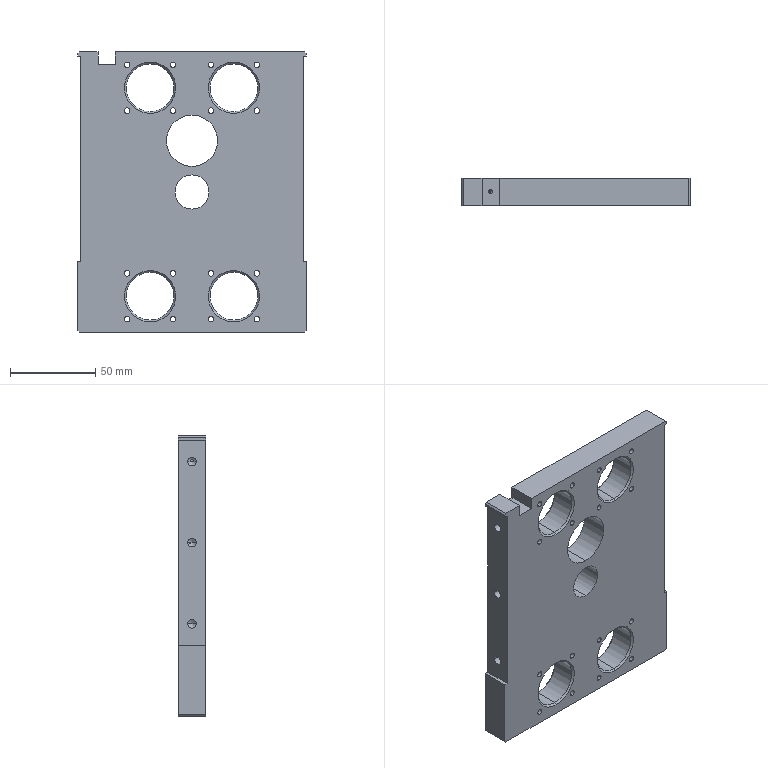Component | SolidWorks | F01AE00111-A2016-1 | 1 solid | 110 faces | box 134 x 16 x 164 mm | volume 282830 mm3 | cylinder 58 | cone 30 | plane 22 | commonest cylinder face diameters 3.3 x32 5 x12 28 x8 2.5 x2 30 x2 20 x2
build123d program:
from build123d import *

# Parameters (mm, degrees)
SKETCH1_W             = 164
SKETCH1_H             = 134
BOSS_EXTRUDE1_DEPTH   = 16
SKETCH2_R             = 14
CUT_EXTRUDE1_DEPTH    = 108.093
M4_TAPPED_HOLE1_D     = 3.3
LPATTERN1_COUNT       = 2
LPATTERN1_PITCH       = 122
LPATTERN1_COUNT_DIR2  = 2
LPATTERN1_PITCH_DIR2  = 49
SKETCH9_R             = 10
CUT_EXTRUDE2_DEPTH    = 108.093
CHAMFER1_SIZE         = 1
M6_TAPPED_HOLE1_D     = 5
M6_TAPPED_HOLE1_DEPTH = 15
M6_TAPPED_HOLE1_TIP   = 1.502
M6_TAPPED_HOLE2_D     = 5
M6_TAPPED_HOLE2_DEPTH = 15
M6_TAPPED_HOLE2_TIP   = 1.502
SKETCH20_W            = 120
SKETCH20_H            = 16
CUT_EXTRUDE3_DEPTH    = 2
SKETCH21_W            = 120
SKETCH21_H            = 16
CUT_EXTRUDE4_DEPTH    = 2
SKETCH22_R            = 15
CUT_EXTRUDE5_DEPTH    = 108.093
CHAMFER2_SIZE         = 1
SKETCH23_W            = 7.2
SKETCH23_H            = 10
CUT_EXTRUDE6_DEPTH    = 108.093
M3_TAPPED_HOLE1_D     = 2.5
M3_TAPPED_HOLE1_DEPTH = 7.5
M3_TAPPED_HOLE1_TIP   = 0.7511


with BuildPart() as part:
    # Sketch1 → Boss-Extrude1 (new body)
    with BuildSketch(Plane.XY):
        Rectangle(SKETCH1_W, SKETCH1_H)
    extrude(amount=BOSS_EXTRUDE1_DEPTH)

    # Sketch2 → Cut-Extrude1 (cut, through all)
    with BuildSketch(Plane.XY.offset(16)):
        with Locations((-61, 24.5)):
            Circle(SKETCH2_R)
        with Locations((-61, -24.5)):
            Circle(SKETCH2_R)
        with Locations((61, 24.5)):
            Circle(SKETCH2_R)
        with Locations((61, -24.5)):
            Circle(SKETCH2_R)
    extrude(amount=-CUT_EXTRUDE1_DEPTH, mode=Mode.SUBTRACT)

    # M4 Tapped Hole1 (through all)
    with Locations(Plane.XY.offset(16)):
        with Locations((-74.435, 37.935), (-47.565, 37.935), (-47.565, 11.065), (-74.435, 11.065), (-61, 24.5)):
            m4_tapped_hole1 = Hole(M4_TAPPED_HOLE1_D / 2)

    # LPattern1: M4 Tapped Hole1 2 × 2
    with Locations(*[(i * LPATTERN1_PITCH, -j * LPATTERN1_PITCH_DIR2, 0) for i in range(LPATTERN1_COUNT) for j in range(LPATTERN1_COUNT_DIR2) if (i, j) != (0, 0)]):
        add(m4_tapped_hole1, mode=Mode.SUBTRACT)

    # Sketch9 → Cut-Extrude2 (cut, through all)
    with BuildSketch(Plane(origin=(0, 0, 0), x_dir=(-1, 0, 0), z_dir=(0, 0, -1))):
        Circle(SKETCH9_R)
    extrude(amount=-CUT_EXTRUDE2_DEPTH, mode=Mode.SUBTRACT)

    # Chamfer1
    chamfer1_edges = [part.edges().sort_by_distance(p)[0] for p in [
        (82, -67, 8),
        (-82, -67, 8),
        (-82, 67, 8),
        (82, 67, 8),
    ]]
    chamfer(chamfer1_edges, length=CHAMFER1_SIZE)

    # M6 Tapped Hole1
    with Locations(Plane(origin=(0, -67, 0), x_dir=(-1, 0, 0), z_dir=(0, -1, 0))):
        with Locations((67, -8), (19.5, -8), (-28, -8)):
            Hole(M6_TAPPED_HOLE1_D / 2, depth=M6_TAPPED_HOLE1_DEPTH)
            with Locations((0, 0, -(M6_TAPPED_HOLE1_DEPTH + M6_TAPPED_HOLE1_TIP / 2))):  # 118° drill point
                Cone(0, M6_TAPPED_HOLE1_D / 2, M6_TAPPED_HOLE1_TIP, mode=Mode.SUBTRACT)

    # M6 Tapped Hole2
    with Locations(Plane(origin=(0, 67, 0), x_dir=(1, 0, 0), z_dir=(0, 1, 0))):
        with Locations((-67, -8), (-19.5, -8), (28, -8)):
            Hole(M6_TAPPED_HOLE2_D / 2, depth=M6_TAPPED_HOLE2_DEPTH)
            with Locations((0, 0, -(M6_TAPPED_HOLE2_DEPTH + M6_TAPPED_HOLE2_TIP / 2))):  # 118° drill point
                Cone(0, M6_TAPPED_HOLE2_D / 2, M6_TAPPED_HOLE2_TIP, mode=Mode.SUBTRACT)

    # Sketch20 → Cut-Extrude3 (cut)
    with BuildSketch(Plane.XZ.offset(67)):
        with Locations((-19.5, 8)):
            Rectangle(SKETCH20_W, SKETCH20_H)
    extrude(amount=-CUT_EXTRUDE3_DEPTH, mode=Mode.SUBTRACT)

    # Sketch21 → Cut-Extrude4 (cut)
    with BuildSketch(Plane(origin=(0, 67, 0), x_dir=(1, 0, 0), z_dir=(0, 1, 0))):
        with Locations((-19.5, -8)):
            Rectangle(SKETCH21_W, SKETCH21_H)
    extrude(amount=-CUT_EXTRUDE4_DEPTH, mode=Mode.SUBTRACT)

    # Sketch22 → Cut-Extrude5 (cut, through all)
    with BuildSketch(Plane(origin=(0, 0, 0), x_dir=(-1, 0, 0), z_dir=(0, 0, -1))):
        with Locations((30, 0)):
            Circle(SKETCH22_R)
    extrude(amount=-CUT_EXTRUDE5_DEPTH, mode=Mode.SUBTRACT)

    # Chamfer2
    chamfer2_edges = [part.edges().sort_by_distance(p)[0] for p in [
        (-75, 24.5, 0),
        (-75, 24.5, 16),
        (-75, -24.5, 0),
        (-75, -24.5, 16),
        (47, 24.5, 0),
        (47, 24.5, 16),
        (47, -24.5, 0),
        (47, -24.5, 16),
    ]]
    chamfer(chamfer2_edges, length=CHAMFER2_SIZE)

    # Sketch23 → Cut-Extrude6 (cut, through all)
    with BuildSketch(Plane.XY.offset(16)):
        with Locations((-78.4, 50)):
            Rectangle(SKETCH23_W, SKETCH23_H)
    extrude(amount=-CUT_EXTRUDE6_DEPTH, mode=Mode.SUBTRACT)

    # M3 Tapped Hole1
    with Locations(Plane(origin=(-74.8, 0.5946, 4.189), x_dir=(0, 0, 1), z_dir=(-1, 0, 0))):
        with Locations((3.811, 49.405)):
            Hole(M3_TAPPED_HOLE1_D / 2, depth=M3_TAPPED_HOLE1_DEPTH)
            with Locations((0, 0, -(M3_TAPPED_HOLE1_DEPTH + M3_TAPPED_HOLE1_TIP / 2))):  # 118° drill point
                Cone(0, M3_TAPPED_HOLE1_D / 2, M3_TAPPED_HOLE1_TIP, mode=Mode.SUBTRACT)


solid = part.part

# Placed as in the assembly
solid = solid.moved(Location((-109.352, -3.452, -272.475), (-90, 0, 90)))